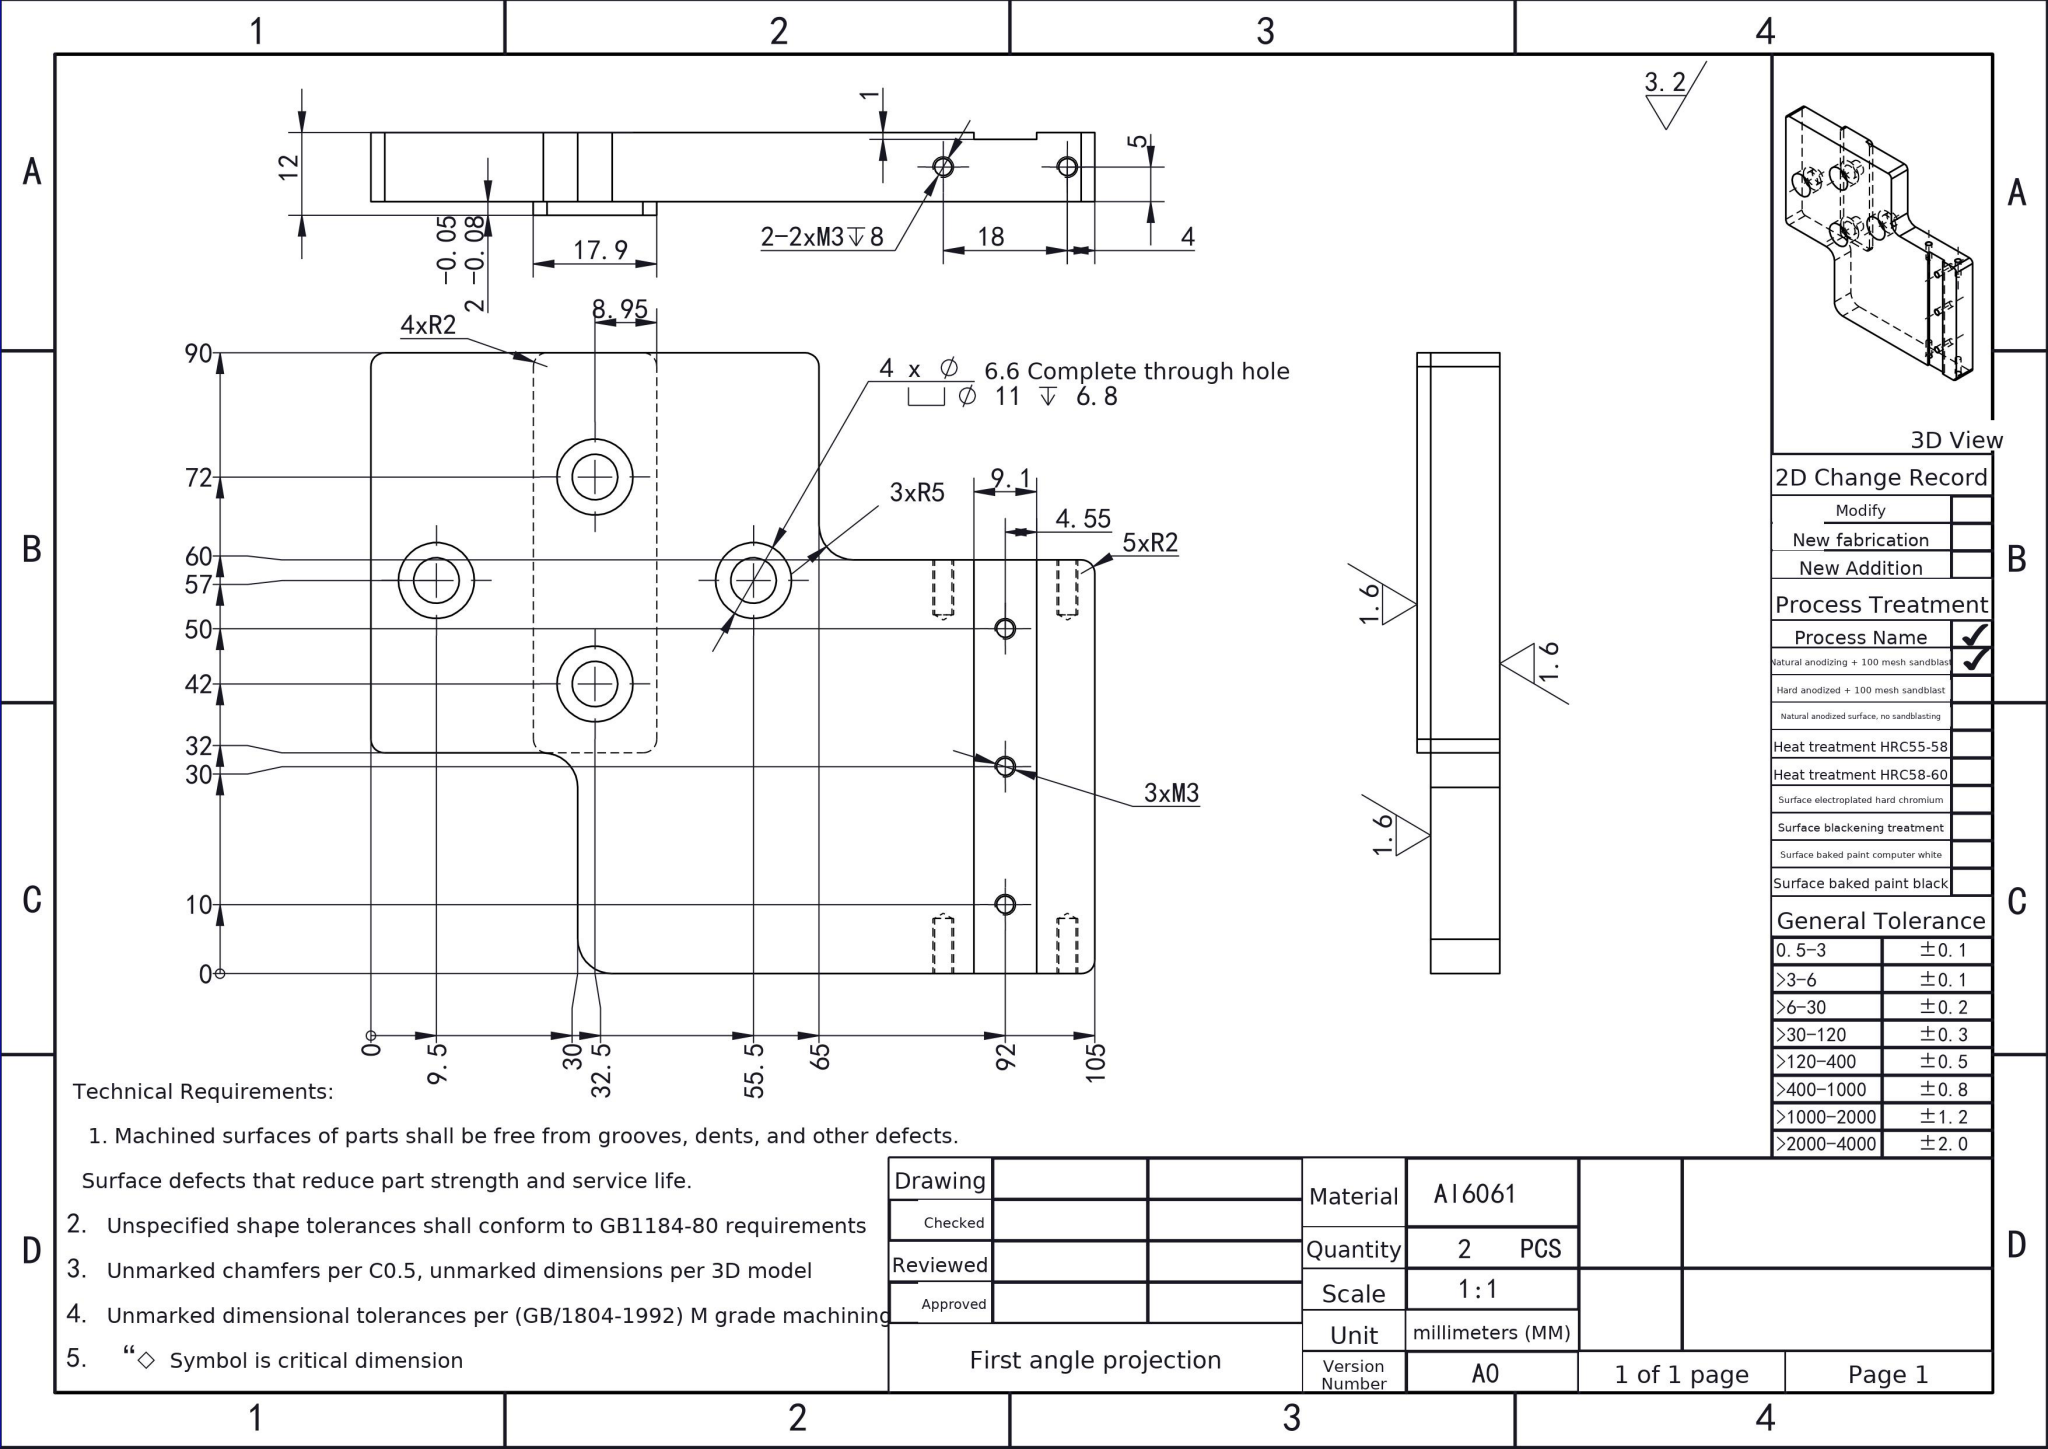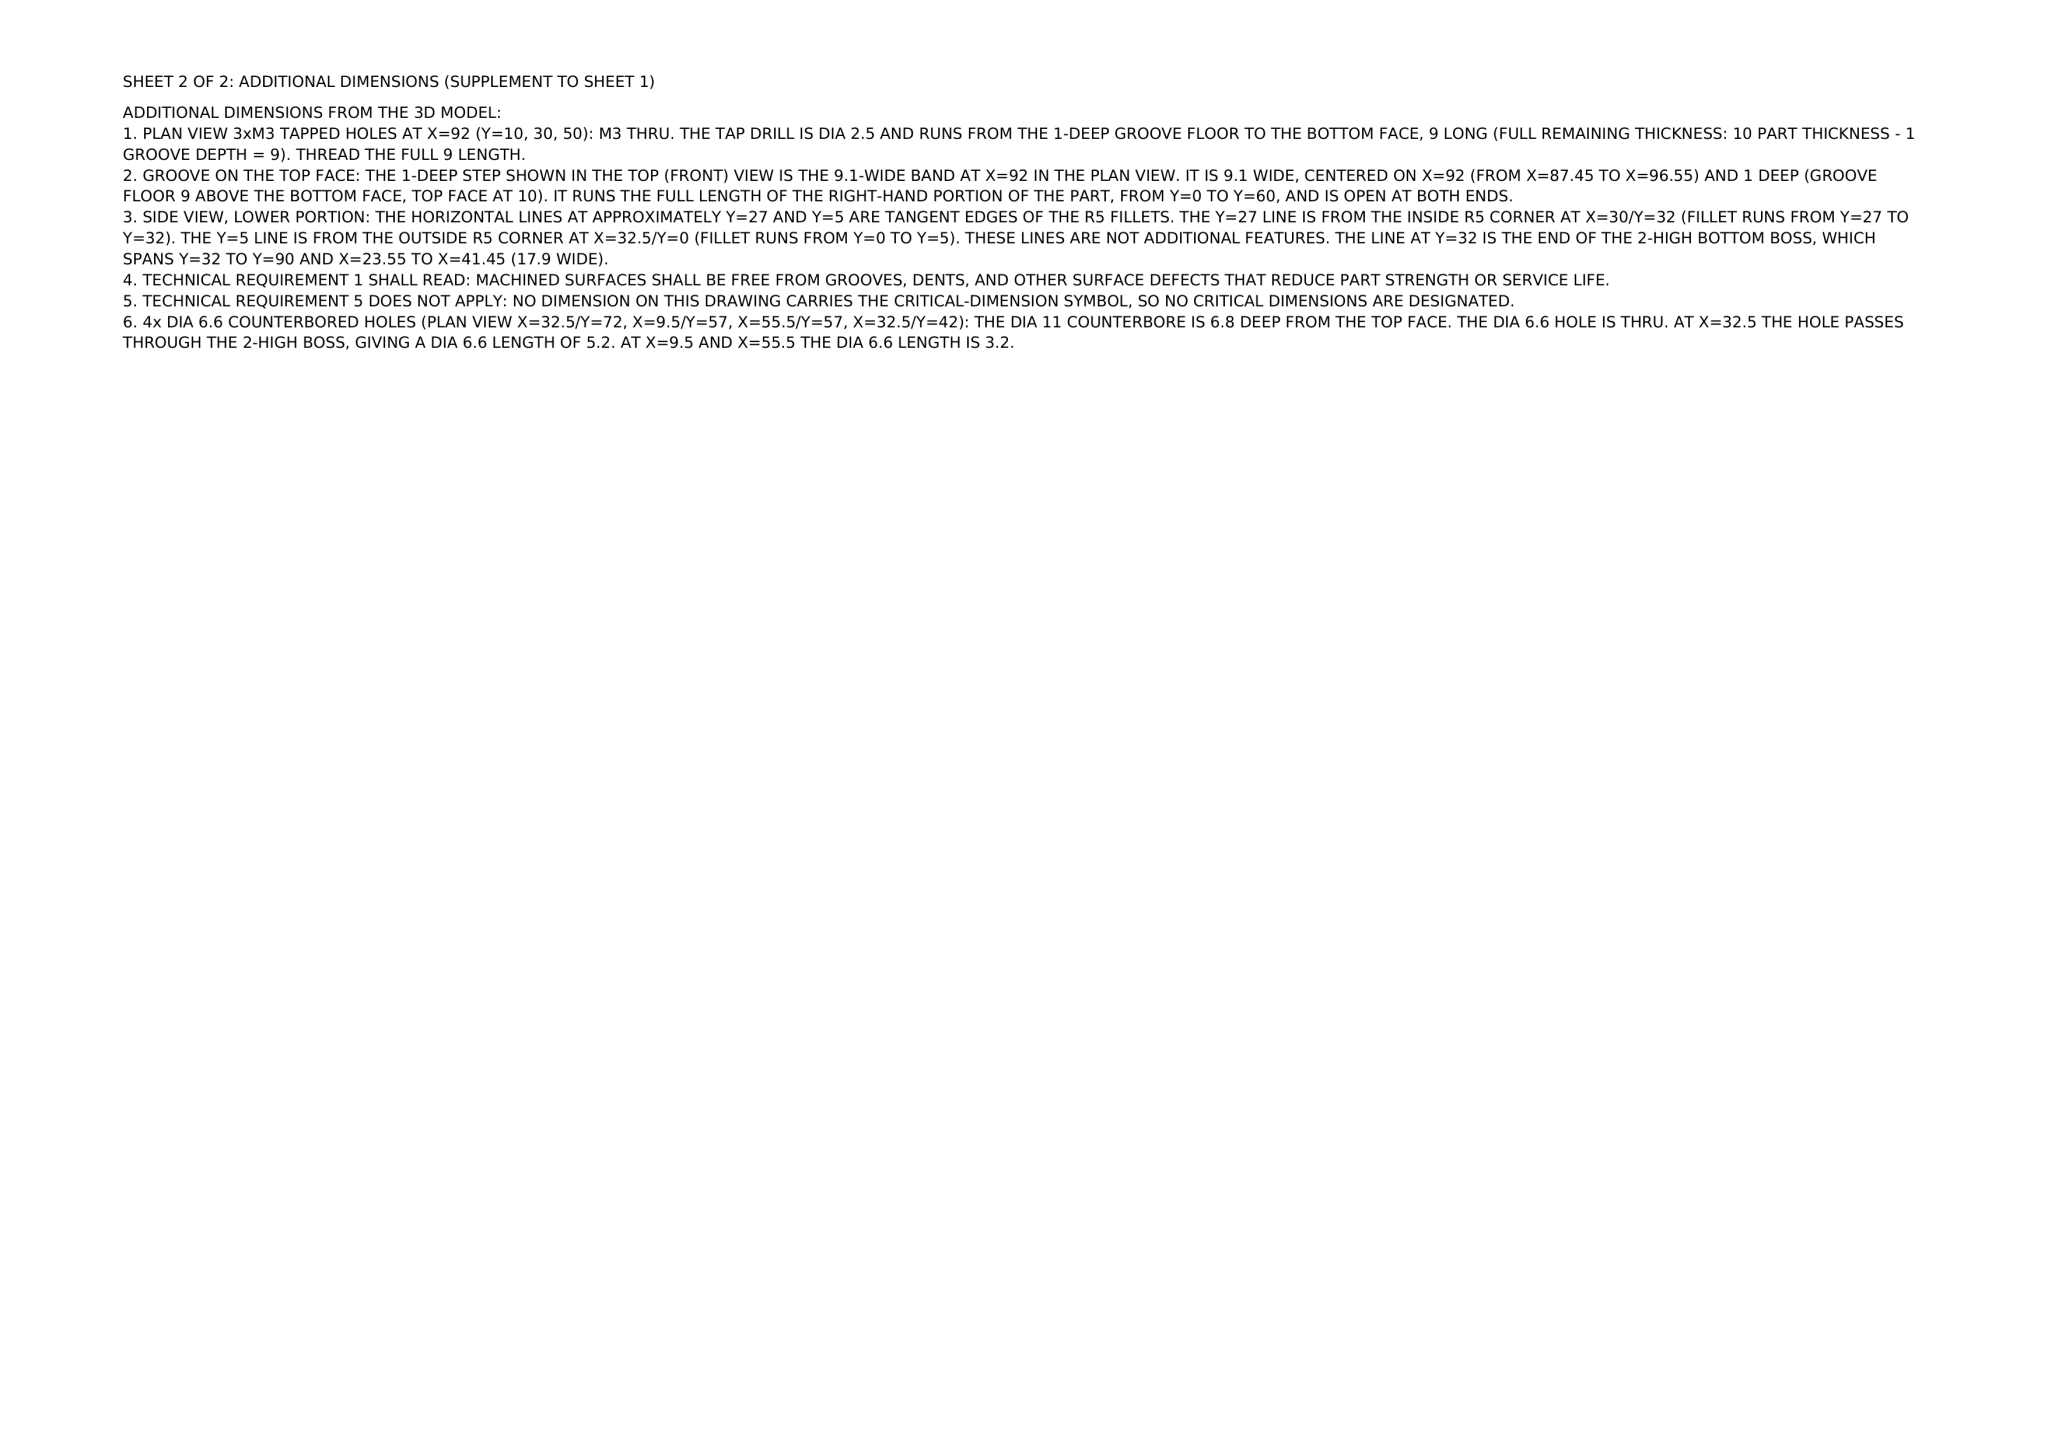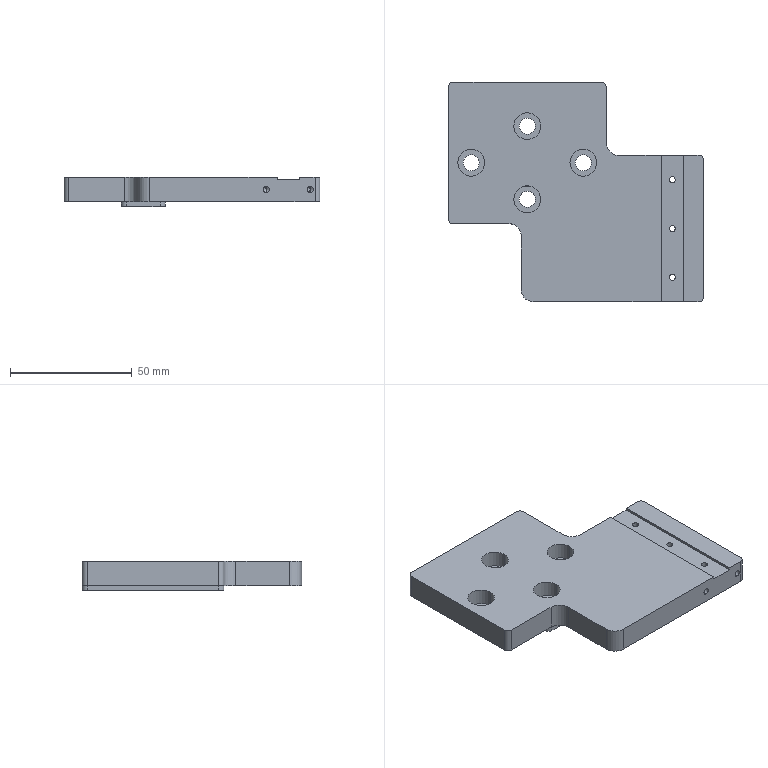Part | NX | mm | Notched Four-Bore Mounting Plate | 1 solid | 73 faces | box 105 x 90 x 12 mm | volume 70980 mm3 | cylinder 42 | plane 23 | cone 8 | commonest cylinder face diameters 2.5 x14 4 x9 11 x8 6.6 x8 10 x3